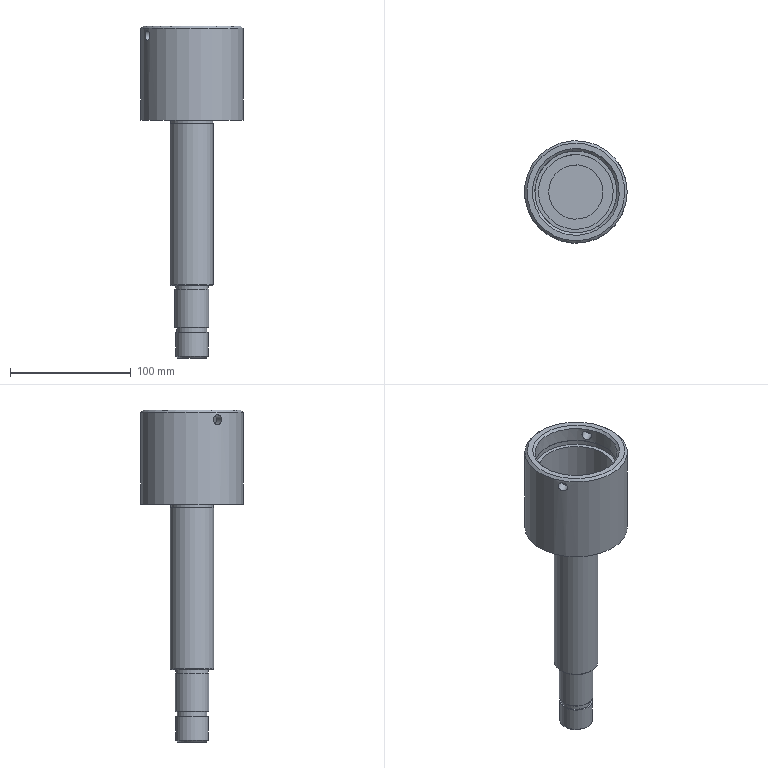Component | NX | PISTON_ROD | 1 solid | 30 faces | volume 415442 mm3 | cylinder 13 | plane 12 | cone 5 | commonest cylinder face diameters 27 x2 8 x2 85 x1 68 x1 24.7 x1 28 x1 36 x1 35 x1